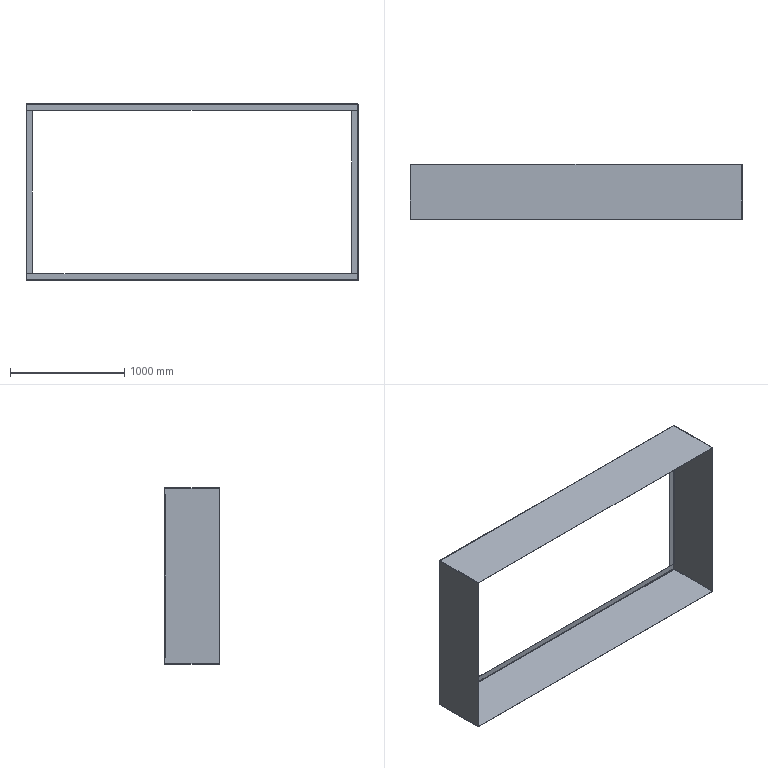Component | NX | BOTTOM_BEAM | 1 solid | 68 faces | volume 9396298 mm3 | plane 54 | cylinder 14 | commonest cylinder face diameters 10 x7 6 x7